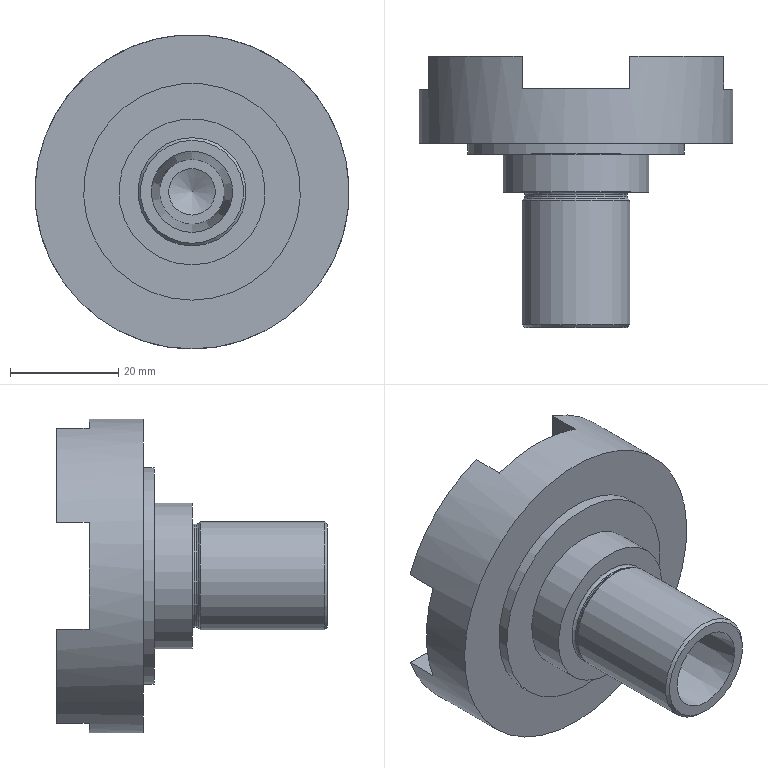Component | NX | GENEVA_SHAFT | 1 solid | 51 faces | volume 33678 mm3 | plane 31 | cylinder 14 | cone 4 | torus 2 | commonest cylinder face diameters 18 x4 6 x4 20 x2 58 x1 40 x1 27 x1 19 x1